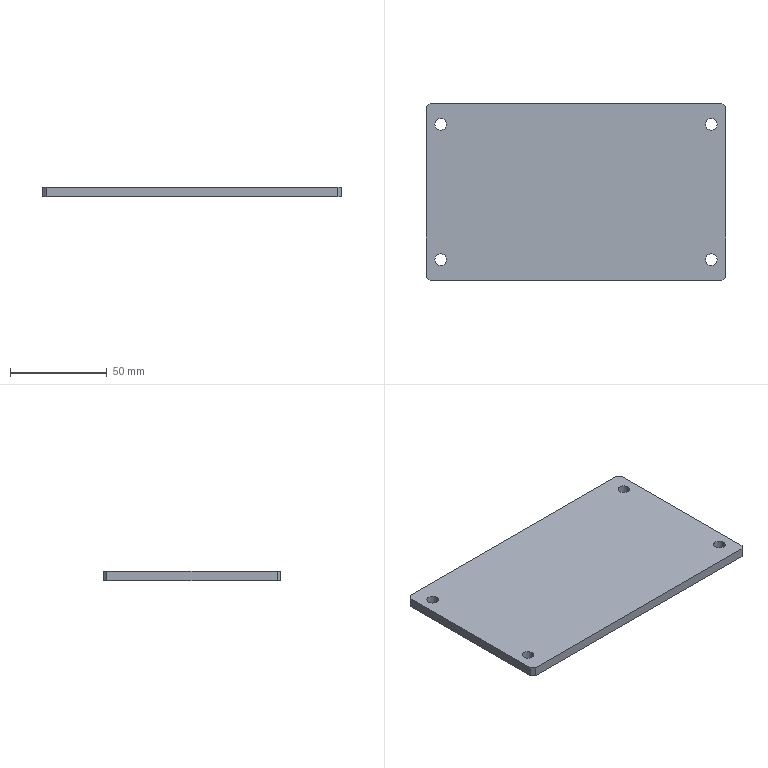CAM job | Mastercam | mm | 4 operations | part box 155 x 92 x 5
1. Helix Bore | 7 - 4 平底刀
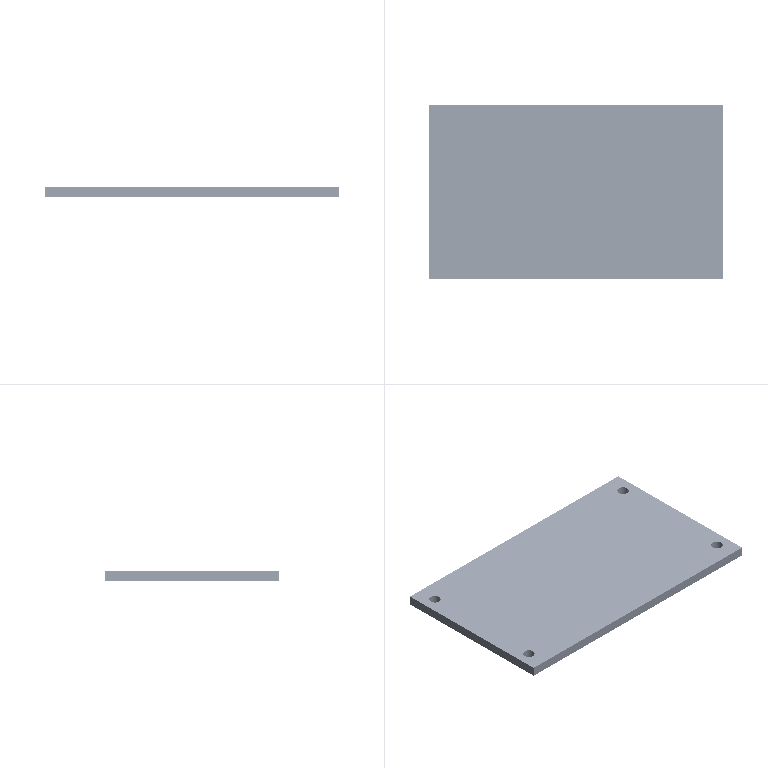2. Contour (Ramp) | 9 - 10C 平底刀
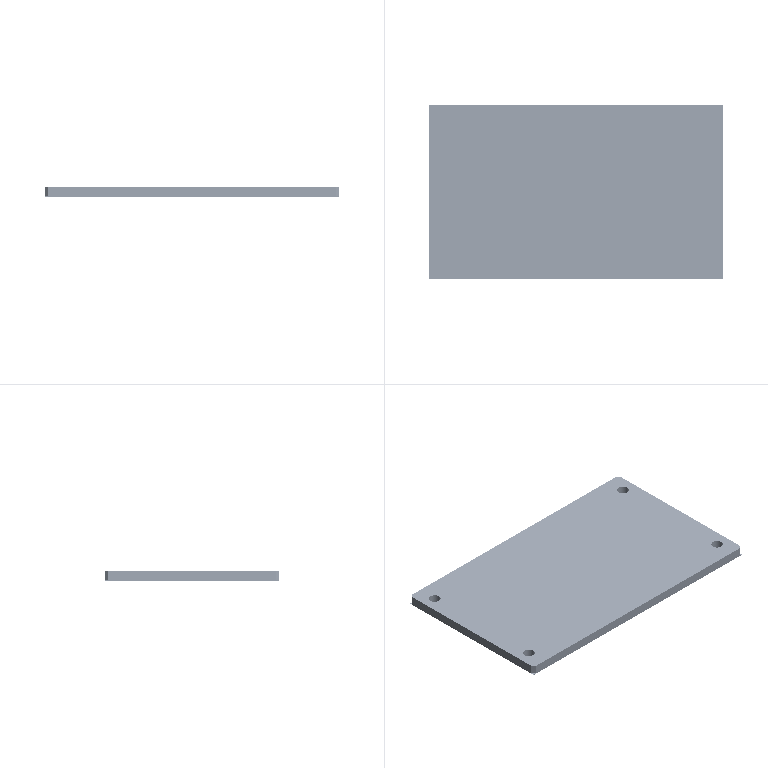3. Contour (2D) | 7 - 4 平底刀
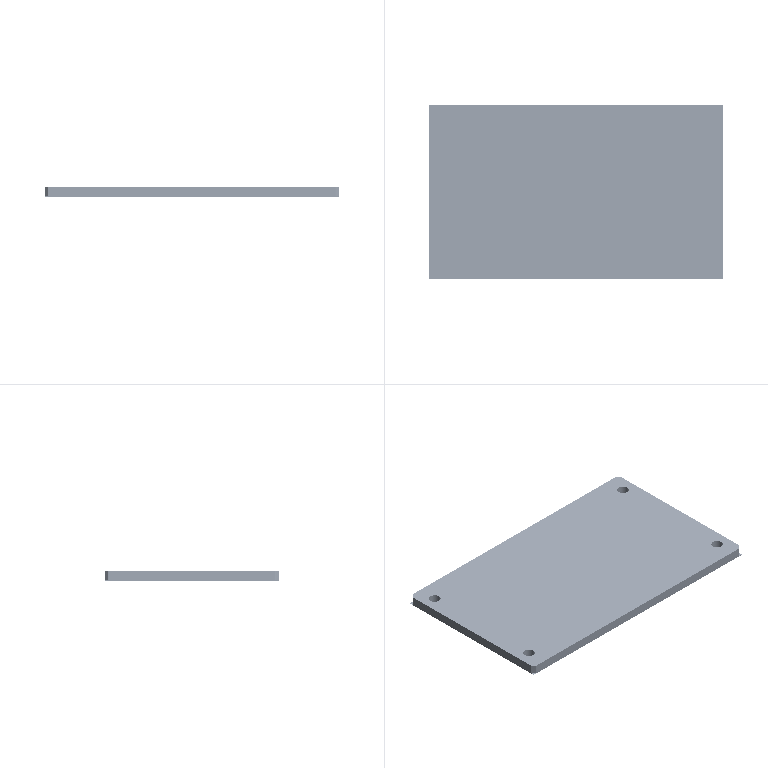4. Model Chamfer | 2 - 6定位倒角